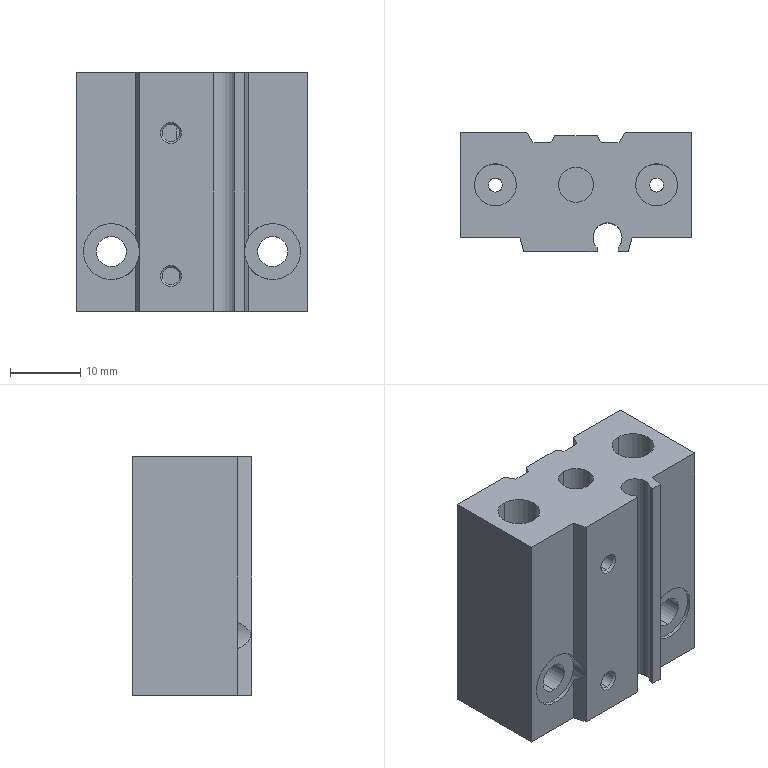Component | SolidWorks | MGJ10-15-1_1-11-1 | 1 solid | 86 faces | volume 13400 mm3 | cylinder 37 | plane 29 | cone 20 | commonest cylinder face diameters 2 x8 3.242 x8 4.3 x4 6 x4 8 x4 2.459 x4 5 x2 10 x2